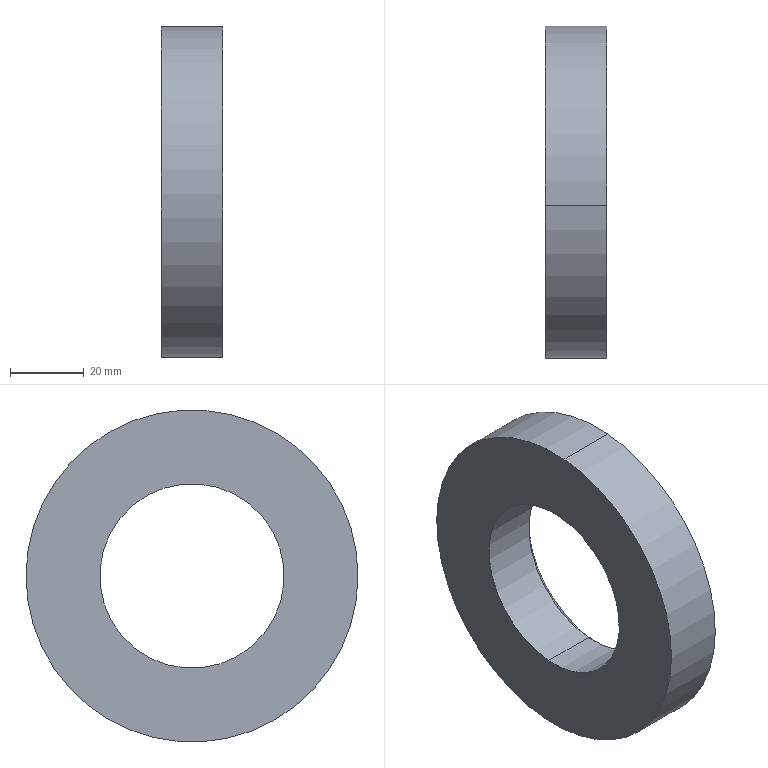Component | SolidWorks | Bearing_2-1 | 1 solid | 8 faces | box 16.79 x 90 x 90 mm | volume 73666 mm3 | cylinder 4 | cone 2 | plane 2 | commonest cylinder face diameters 50 x2 90 x2
build123d program:
from build123d import *

# Parameters (mm, degrees)
SKETCH1_R           = 45
SKETCH1_R_2         = 25
BOSS_EXTRUDE1_DEPTH = 16.79
CHAMFER1_SIZE       = 1.5


with BuildPart() as part:
    # Sketch1 → Boss-Extrude1 (new body)
    with BuildSketch(Plane(origin=(0, 0, 0), x_dir=(0, 0, -1), z_dir=(1, 0, 0))):
        Circle(SKETCH1_R)
        Circle(SKETCH1_R_2, mode=Mode.SUBTRACT)
    extrude(amount=BOSS_EXTRUDE1_DEPTH)

    # Chamfer1
    chamfer1_edges = [part.edges().sort_by_distance(p)[0] for p in [
        (16.79, 0, 25),
    ]]
    chamfer(chamfer1_edges, length=CHAMFER1_SIZE)


solid = part.part

# Placed as in the assembly
solid = solid.moved(Location((602.733, 15.31, -110), (0, 0, 0)))
STEP:
#1=CARTESIAN_POINT('',(24.332,0.5199,-3.35));
#2=VERTEX_POINT('',#1);
#3=CARTESIAN_POINT('',(24.332,0.6856,-5.311));
#4=VERTEX_POINT('',#3);
#5=CARTESIAN_POINT('',(24.332,0.6028,-4.331));
#6=DIRECTION('',(1.,0.,0.));
#7=DIRECTION('',(0.,0.08416,-0.9965));
#8=AXIS2_PLACEMENT_3D('',#5,#6,#7);
#9=CIRCLE('',#8,0.9843);
#10=EDGE_CURVE('',#2,#4,#9,.T.);
#11=ORIENTED_EDGE('',*,*,#10,.F.);
#12=CARTESIAN_POINT('',(24.391,0.515,-3.291));
#13=VERTEX_POINT('',#12);
#14=CARTESIAN_POINT('',(24.332,0.5199,-3.35));
#15=DIRECTION('',(0.7071,-0.05951,0.7046));
#16=VECTOR('',#15,39.37);
#17=LINE('',#14,#16);
#18=EDGE_CURVE('',#2,#13,#17,.T.);
#19=ORIENTED_EDGE('',*,*,#18,.T.);
#20=CARTESIAN_POINT('',(24.391,0.6906,-5.37));
#21=VERTEX_POINT('',#20);
#22=CARTESIAN_POINT('',(24.391,0.6028,-4.331));
#23=DIRECTION('',(-1.,0.,0.));
#24=DIRECTION('',(0.,0.08416,-0.9965));
#25=AXIS2_PLACEMENT_3D('',#22,#23,#24);
#26=CIRCLE('',#25,1.043);
#27=EDGE_CURVE('',#21,#13,#26,.T.);
#28=ORIENTED_EDGE('',*,*,#27,.F.);
#29=CARTESIAN_POINT('',(24.332,0.6856,-5.311));
#30=DIRECTION('',(0.7071,0.05951,-0.7046));
#31=VECTOR('',#30,39.37);
#32=LINE('',#29,#31);
#33=EDGE_CURVE('',#4,#21,#32,.T.);
#34=ORIENTED_EDGE('',*,*,#33,.F.);
#35=EDGE_LOOP('',(#11,#19,#28,#34));
#36=FACE_OUTER_BOUND('',#35,.T.);
#37=CARTESIAN_POINT('',(24.332,0.6028,-4.331));
#38=DIRECTION('',(1.,0.,0.));
#39=DIRECTION('',(0.,0.08416,-0.9965));
#40=AXIS2_PLACEMENT_3D('',#37,#38,#39);
#41=CONICAL_SURFACE('',#40,0.9843,0.7854);
#42=ADVANCED_FACE('',(#36),#41,.F.);
#43=ORIENTED_EDGE('',*,*,#10,.T.);
#44=CARTESIAN_POINT('',(23.73,0.6856,-5.311));
#45=VERTEX_POINT('',#44);
#46=CARTESIAN_POINT('',(24.391,0.6856,-5.311));
#47=DIRECTION('',(-1.,0.,0.));
#48=VECTOR('',#47,39.37);
#49=LINE('',#46,#48);
#50=EDGE_CURVE('',#4,#45,#49,.T.);
#51=ORIENTED_EDGE('',*,*,#50,.T.);
#52=CARTESIAN_POINT('',(23.73,0.5199,-3.35));
#53=VERTEX_POINT('',#52);
#54=CARTESIAN_POINT('',(23.73,0.6028,-4.331));
#55=DIRECTION('',(1.,0.,0.));
#56=DIRECTION('',(0.,0.08416,-0.9965));
#57=AXIS2_PLACEMENT_3D('',#54,#55,#56);
#58=CIRCLE('',#57,0.9843);
#59=EDGE_CURVE('',#53,#45,#58,.T.);
#60=ORIENTED_EDGE('',*,*,#59,.F.);
#61=CARTESIAN_POINT('',(24.391,0.5199,-3.35));
#62=DIRECTION('',(-1.,0.,0.));
#63=VECTOR('',#62,39.37);
#64=LINE('',#61,#63);
#65=EDGE_CURVE('',#2,#53,#64,.T.);
#66=ORIENTED_EDGE('',*,*,#65,.F.);
#67=EDGE_LOOP('',(#43,#51,#60,#66));
#68=FACE_OUTER_BOUND('',#67,.T.);
#69=CARTESIAN_POINT('',(24.391,0.6028,-4.331));
#70=DIRECTION('',(-1.,0.,0.));
#71=DIRECTION('',(0.,-0.08416,0.9965));
#72=AXIS2_PLACEMENT_3D('',#69,#70,#71);
#73=CYLINDRICAL_SURFACE('',#72,0.9843);
#74=ADVANCED_FACE('',(#68),#73,.F.);
#75=CARTESIAN_POINT('',(24.391,0.7519,-6.096));
#76=VERTEX_POINT('',#75);
#77=CARTESIAN_POINT('',(24.391,0.4537,-2.565));
#78=VERTEX_POINT('',#77);
#79=CARTESIAN_POINT('',(24.391,0.6028,-4.331));
#80=DIRECTION('',(1.,0.,0.));
#81=DIRECTION('',(0.,0.08416,-0.9965));
#82=AXIS2_PLACEMENT_3D('',#79,#80,#81);
#83=CIRCLE('',#82,1.772);
#84=EDGE_CURVE('',#76,#78,#83,.T.);
#85=ORIENTED_EDGE('',*,*,#84,.F.);
#86=CARTESIAN_POINT('',(23.73,0.7519,-6.096));
#87=VERTEX_POINT('',#86);
#88=CARTESIAN_POINT('',(24.391,0.7519,-6.096));
#89=DIRECTION('',(-1.,0.,0.));
#90=VECTOR('',#89,39.37);
#91=LINE('',#88,#90);
#92=EDGE_CURVE('',#76,#87,#91,.T.);
#93=ORIENTED_EDGE('',*,*,#92,.T.);
#94=CARTESIAN_POINT('',(23.73,0.4537,-2.565));
#95=VERTEX_POINT('',#94);
#96=CARTESIAN_POINT('',(23.73,0.6028,-4.331));
#97=DIRECTION('',(1.,0.,0.));
#98=DIRECTION('',(0.,0.08416,-0.9965));
#99=AXIS2_PLACEMENT_3D('',#96,#97,#98);
#100=CIRCLE('',#99,1.772);
#101=EDGE_CURVE('',#87,#95,#100,.T.);
#102=ORIENTED_EDGE('',*,*,#101,.T.);
#103=CARTESIAN_POINT('',(24.391,0.4537,-2.565));
#104=DIRECTION('',(-1.,0.,0.));
#105=VECTOR('',#104,39.37);
#106=LINE('',#103,#105);
#107=EDGE_CURVE('',#78,#95,#106,.T.);
#108=ORIENTED_EDGE('',*,*,#107,.F.);
#109=EDGE_LOOP('',(#85,#93,#102,#108));
#110=FACE_OUTER_BOUND('',#109,.T.);
#111=CARTESIAN_POINT('',(24.391,0.6028,-4.331));
#112=DIRECTION('',(-1.,0.,0.));
#113=DIRECTION('',(0.,-0.08416,0.9965));
#114=AXIS2_PLACEMENT_3D('',#111,#112,#113);
#115=CYLINDRICAL_SURFACE('',#114,1.772);
#116=ADVANCED_FACE('',(#110),#115,.T.);
#117=ORIENTED_EDGE('',*,*,#27,.T.);
#118=CARTESIAN_POINT('',(24.391,0.6028,-4.331));
#119=DIRECTION('',(-1.,0.,0.));
#120=DIRECTION('',(0.,0.08416,-0.9965));
#121=AXIS2_PLACEMENT_3D('',#118,#119,#120);
#122=CIRCLE('',#121,1.043);
#123=EDGE_CURVE('',#13,#21,#122,.T.);
#124=ORIENTED_EDGE('',*,*,#123,.T.);
#125=EDGE_LOOP('',(#117,#124));
#126=FACE_BOUND('',#125,.T.);
#127=CARTESIAN_POINT('',(24.391,0.6028,-4.331));
#128=DIRECTION('',(1.,0.,0.));
#129=DIRECTION('',(0.,0.08416,-0.9965));
#130=AXIS2_PLACEMENT_3D('',#127,#128,#129);
#131=CIRCLE('',#130,1.772);
#132=EDGE_CURVE('',#78,#76,#131,.T.);
#133=ORIENTED_EDGE('',*,*,#132,.T.);
#134=ORIENTED_EDGE('',*,*,#84,.T.);
#135=EDGE_LOOP('',(#133,#134));
#136=FACE_OUTER_BOUND('',#135,.T.);
#137=CARTESIAN_POINT('',(24.391,0.6028,-4.331));
#138=DIRECTION('',(1.,0.,0.));
#139=DIRECTION('',(0.,0.08416,-0.9965));
#140=AXIS2_PLACEMENT_3D('',#137,#138,#139);
#141=PLANE('',#140);
#142=ADVANCED_FACE('',(#126,#136),#141,.T.);
#143=CARTESIAN_POINT('',(23.73,0.6028,-4.331));
#144=DIRECTION('',(1.,0.,0.));
#145=DIRECTION('',(0.,0.08416,-0.9965));
#146=AXIS2_PLACEMENT_3D('',#143,#144,#145);
#147=CIRCLE('',#146,1.772);
#148=EDGE_CURVE('',#95,#87,#147,.T.);
#149=ORIENTED_EDGE('',*,*,#148,.F.);
#150=ORIENTED_EDGE('',*,*,#101,.F.);
#151=EDGE_LOOP('',(#149,#150));
#152=FACE_OUTER_BOUND('',#151,.T.);
#153=ORIENTED_EDGE('',*,*,#59,.T.);
#154=CARTESIAN_POINT('',(23.73,0.6028,-4.331));
#155=DIRECTION('',(1.,0.,0.));
#156=DIRECTION('',(0.,0.08416,-0.9965));
#157=AXIS2_PLACEMENT_3D('',#154,#155,#156);
#158=CIRCLE('',#157,0.9843);
#159=EDGE_CURVE('',#45,#53,#158,.T.);
#160=ORIENTED_EDGE('',*,*,#159,.T.);
#161=EDGE_LOOP('',(#153,#160));
#162=FACE_BOUND('',#161,.T.);
#163=CARTESIAN_POINT('',(23.73,0.6028,-4.331));
#164=DIRECTION('',(1.,0.,0.));
#165=DIRECTION('',(0.,0.08416,-0.9965));
#166=AXIS2_PLACEMENT_3D('',#163,#164,#165);
#167=PLANE('',#166);
#168=ADVANCED_FACE('',(#152,#162),#167,.F.);
#169=ORIENTED_EDGE('',*,*,#92,.F.);
#170=ORIENTED_EDGE('',*,*,#132,.F.);
#171=ORIENTED_EDGE('',*,*,#107,.T.);
#172=ORIENTED_EDGE('',*,*,#148,.T.);
#173=EDGE_LOOP('',(#169,#170,#171,#172));
#174=FACE_OUTER_BOUND('',#173,.T.);
#175=CARTESIAN_POINT('',(24.391,0.6028,-4.331));
#176=DIRECTION('',(-1.,0.,0.));
#177=DIRECTION('',(0.,-0.08416,0.9965));
#178=AXIS2_PLACEMENT_3D('',#175,#176,#177);
#179=CYLINDRICAL_SURFACE('',#178,1.772);
#180=ADVANCED_FACE('',(#174),#179,.T.);
#181=ORIENTED_EDGE('',*,*,#50,.F.);
#182=CARTESIAN_POINT('',(24.332,0.6028,-4.331));
#183=DIRECTION('',(1.,0.,0.));
#184=DIRECTION('',(0.,0.08416,-0.9965));
#185=AXIS2_PLACEMENT_3D('',#182,#183,#184);
#186=CIRCLE('',#185,0.9843);
#187=EDGE_CURVE('',#4,#2,#186,.T.);
#188=ORIENTED_EDGE('',*,*,#187,.T.);
#189=ORIENTED_EDGE('',*,*,#65,.T.);
#190=ORIENTED_EDGE('',*,*,#159,.F.);
#191=EDGE_LOOP('',(#181,#188,#189,#190));
#192=FACE_OUTER_BOUND('',#191,.T.);
#193=CARTESIAN_POINT('',(24.391,0.6028,-4.331));
#194=DIRECTION('',(-1.,0.,0.));
#195=DIRECTION('',(0.,-0.08416,0.9965));
#196=AXIS2_PLACEMENT_3D('',#193,#194,#195);
#197=CYLINDRICAL_SURFACE('',#196,0.9843);
#198=ADVANCED_FACE('',(#192),#197,.F.);
#199=ORIENTED_EDGE('',*,*,#18,.F.);
#200=ORIENTED_EDGE('',*,*,#187,.F.);
#201=ORIENTED_EDGE('',*,*,#33,.T.);
#202=ORIENTED_EDGE('',*,*,#123,.F.);
#203=EDGE_LOOP('',(#199,#200,#201,#202));
#204=FACE_OUTER_BOUND('',#203,.T.);
#205=CARTESIAN_POINT('',(24.332,0.6028,-4.331));
#206=DIRECTION('',(1.,0.,0.));
#207=DIRECTION('',(0.,0.08416,-0.9965));
#208=AXIS2_PLACEMENT_3D('',#205,#206,#207);
#209=CONICAL_SURFACE('',#208,0.9843,0.7854);
#210=ADVANCED_FACE('',(#204),#209,.F.);
#211=CLOSED_SHELL('',(#42,#74,#116,#142,#168,#180,#198,#210));
#212=MANIFOLD_SOLID_BREP('',#211);
#213=CARTESIAN_POINT('',(0.,0.,0.));
#214=DIRECTION('',(0.,0.,1.));
#215=DIRECTION('',(1.,0.,0.));
#216=AXIS2_PLACEMENT_3D('',#213,#214,#215);
#217=(LENGTH_UNIT()NAMED_UNIT(*)SI_UNIT($,.METRE.));
#218=LENGTH_MEASURE_WITH_UNIT(LENGTH_MEASURE(0.0254),#217);
#219=DIMENSIONAL_EXPONENTS(1.,0.,0.,0.,0.,0.,0.);
#220=(CONVERSION_BASED_UNIT('',#218)LENGTH_UNIT()NAMED_UNIT(#219));
#221=UNCERTAINTY_MEASURE_WITH_UNIT(LENGTH_MEASURE(0.00001),#220,'','');
#222=(NAMED_UNIT(*)PLANE_ANGLE_UNIT()SI_UNIT($,.RADIAN.));
#223=(NAMED_UNIT(*)SI_UNIT($,.STERADIAN.)SOLID_ANGLE_UNIT());
#224=(GEOMETRIC_REPRESENTATION_CONTEXT(3)GLOBAL_UNCERTAINTY_ASSIGNED_CONTEXT((#221))GLOBAL_UNIT_ASSIGNED_CONTEXT((#220,#222,#223))REPRESENTATION_CONTEXT('',''));
#225=ADVANCED_BREP_SHAPE_REPRESENTATION('',(#212,#216),#224);
#226=COLOUR_RGB('',0.7922,0.8196,0.9333);
#227=FILL_AREA_STYLE_COLOUR('',#226);
#228=FILL_AREA_STYLE('',(#227));
#229=SURFACE_STYLE_FILL_AREA(#228);
#230=SURFACE_SIDE_STYLE('',(#229));
#231=SURFACE_STYLE_USAGE(.BOTH.,#230);
#232=PRESENTATION_STYLE_ASSIGNMENT((#231));
#233=STYLED_ITEM('',(#232),#212);
#234=PRESENTATION_LAYER_ASSIGNMENT('','',(#233));
#235=(LENGTH_UNIT()NAMED_UNIT(*)SI_UNIT($,.METRE.));
#236=LENGTH_MEASURE_WITH_UNIT(LENGTH_MEASURE(0.0254),#235);
#237=DIMENSIONAL_EXPONENTS(1.,0.,0.,0.,0.,0.,0.);
#238=(CONVERSION_BASED_UNIT('',#236)LENGTH_UNIT()NAMED_UNIT(#237));
#239=UNCERTAINTY_MEASURE_WITH_UNIT(LENGTH_MEASURE(0.00001),#238,'','');
#240=(NAMED_UNIT(*)PLANE_ANGLE_UNIT()SI_UNIT($,.RADIAN.));
#241=(NAMED_UNIT(*)SI_UNIT($,.STERADIAN.)SOLID_ANGLE_UNIT());
#242=(GEOMETRIC_REPRESENTATION_CONTEXT(3)GLOBAL_UNCERTAINTY_ASSIGNED_CONTEXT((#239))GLOBAL_UNIT_ASSIGNED_CONTEXT((#238,#240,#241))REPRESENTATION_CONTEXT('',''));
#243=MECHANICAL_DESIGN_GEOMETRIC_PRESENTATION_REPRESENTATION('',(#233),#242);